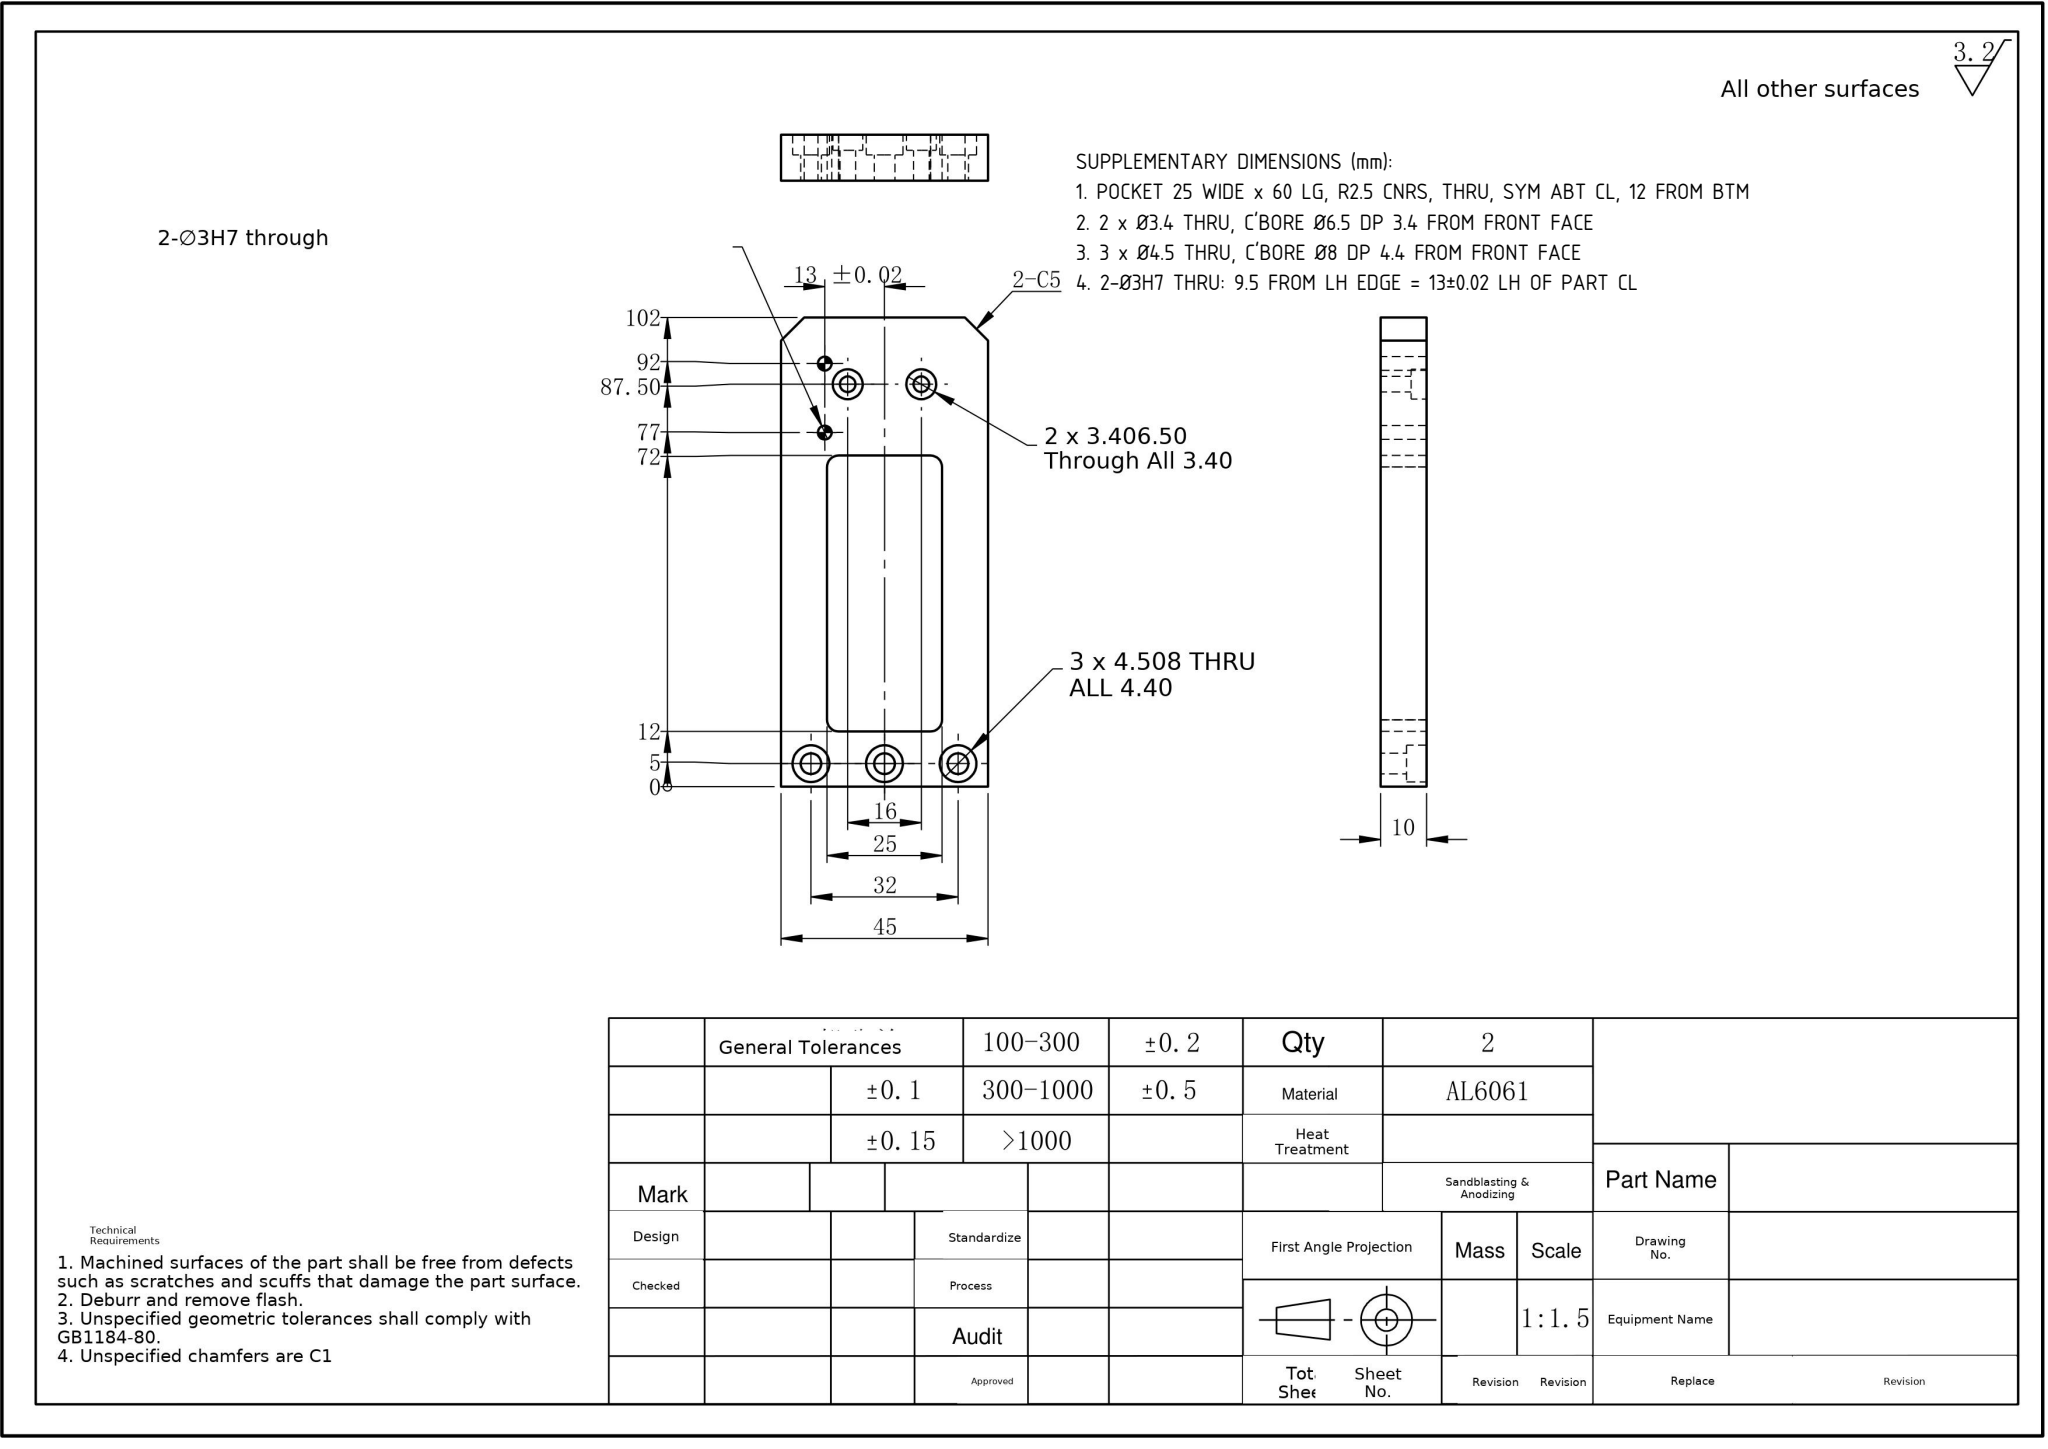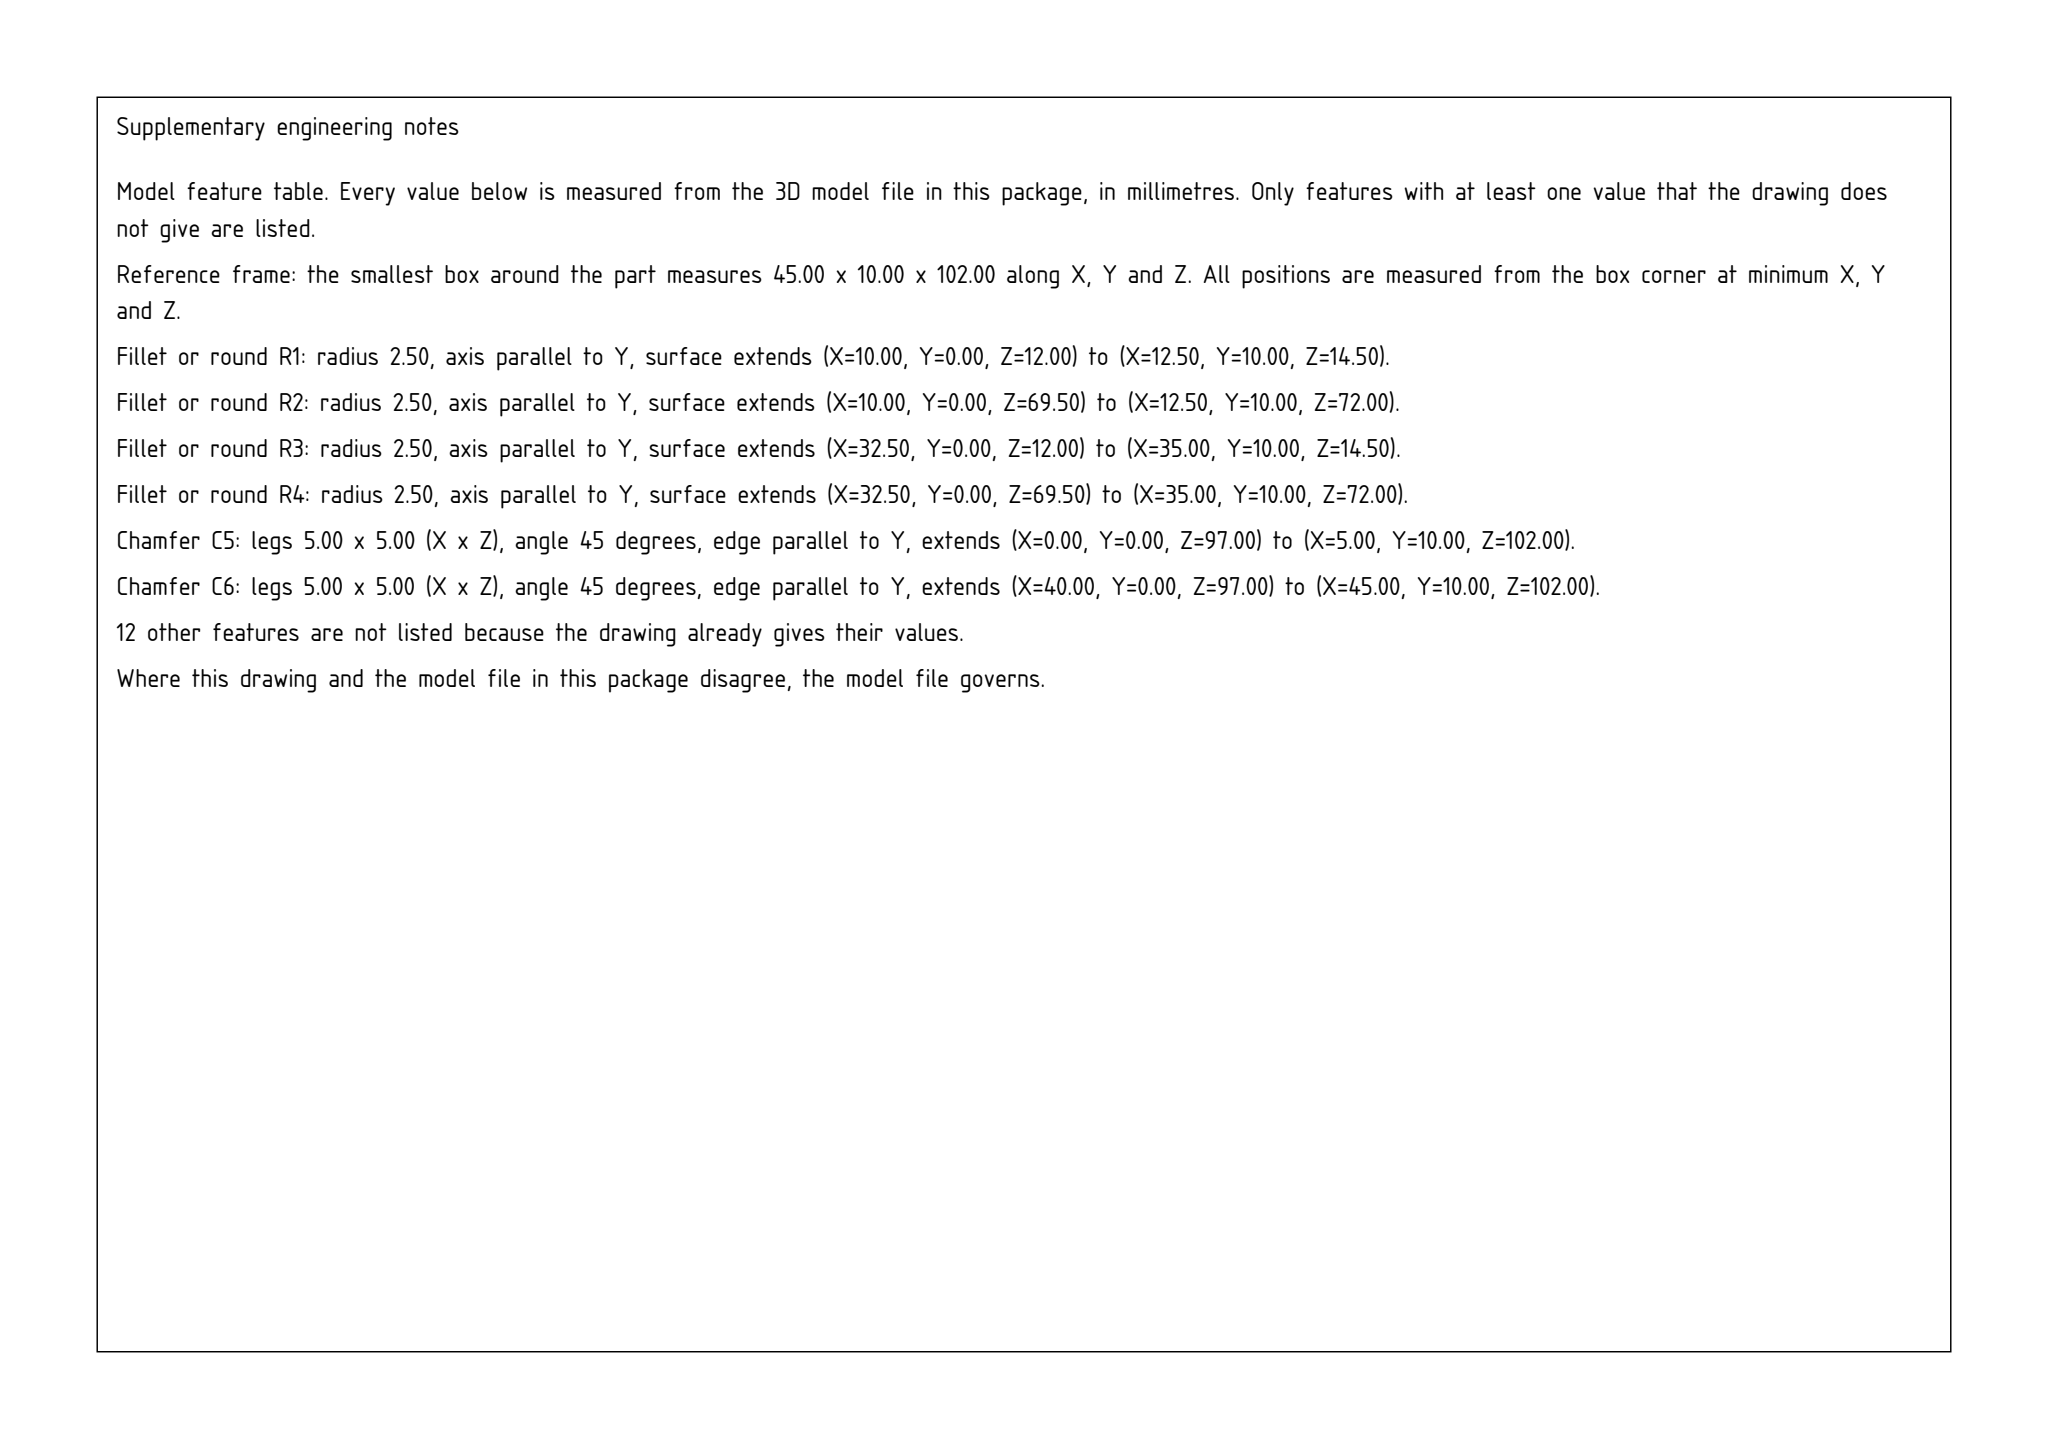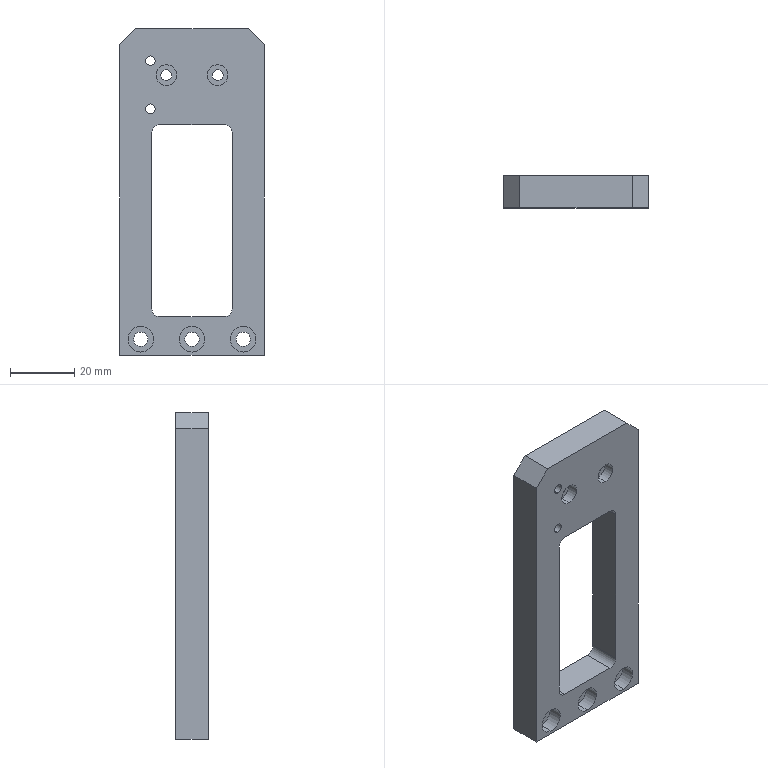Part | SolidWorks | mm | 1 solid | 45 faces | box 45 x 10 x 102 mm | volume 29286 mm3 | cylinder 28 | plane 17 | commonest cylinder face diameters 8 x6 4.5 x6 3 x4 6.5 x4 3.4 x4 5 x4
build123d program:
from build123d import *

# Parameters (mm, degrees)
SKETCH1_W                                       = 45
SKETCH1_H                                       = 102
BOSS_EXTRUDE1_DEPTH                             = 5
M4_HEX_SOCKET_HEAD_CAP_SCREW_CBORE1_D           = 4.5
M4_HEX_SOCKET_HEAD_CAP_SCREW_CBORE1_CBORE_D     = 8
M4_HEX_SOCKET_HEAD_CAP_SCREW_CBORE1_CBORE_DEPTH = 4.4
CHAMFER1_SIZE                                   = 5
M3_HEX_SOCKET_HEAD_CAP_SCREW_CBORE1_D           = 3.4
M3_HEX_SOCKET_HEAD_CAP_SCREW_CBORE1_CBORE_D     = 6.5
M3_HEX_SOCKET_HEAD_CAP_SCREW_CBORE1_CBORE_DEPTH = 3.4
SKETCH6_W                                       = 25
SKETCH6_H                                       = 60
CUT_EXTRUDE1_DEPTH                              = 10
FILLET1_R                                       = 2.5
SKETCH7_R                                       = 1.5
CUT_EXTRUDE2_DEPTH                              = 10


with BuildPart() as part:
    # Sketch1 → Boss-Extrude1 (new, symmetric)
    with BuildSketch(Plane(origin=(0, 0, 0), x_dir=(1, 0, 0), z_dir=(0, 1, 0))):
        Rectangle(SKETCH1_W, SKETCH1_H)
    extrude(amount=BOSS_EXTRUDE1_DEPTH, both=True)

    # M4 Hex Socket Head Cap Screw CBORE1 (through all)
    with Locations(Plane(origin=(0, -5, 0), x_dir=(-1, 0, 0), z_dir=(0, -1, 0))):
        with Locations((0, 46), (16, 46), (-16, 46)):
            CounterBoreHole(M4_HEX_SOCKET_HEAD_CAP_SCREW_CBORE1_D / 2, M4_HEX_SOCKET_HEAD_CAP_SCREW_CBORE1_CBORE_D / 2, M4_HEX_SOCKET_HEAD_CAP_SCREW_CBORE1_CBORE_DEPTH)

    # Chamfer1
    chamfer1_edges = [part.edges().sort_by_distance(p)[0] for p in [
        (22.5, 0, 51),
        (-22.5, 0, 51),
    ]]
    chamfer(chamfer1_edges, length=CHAMFER1_SIZE)

    # M3 Hex Socket Head Cap Screw CBORE1 (through all)
    with Locations(Plane(origin=(0, -5, 0), x_dir=(-1, 0, 0), z_dir=(0, -1, 0))):
        with Locations((-8, -36.5), (8, -36.5)):
            CounterBoreHole(M3_HEX_SOCKET_HEAD_CAP_SCREW_CBORE1_D / 2, M3_HEX_SOCKET_HEAD_CAP_SCREW_CBORE1_CBORE_D / 2, M3_HEX_SOCKET_HEAD_CAP_SCREW_CBORE1_CBORE_DEPTH)

    # Sketch6 → Cut-Extrude1 (cut)
    with BuildSketch(Plane(origin=(0, 5, 0), x_dir=(1, 0, 0), z_dir=(0, 1, 0))):
        with Locations((0, 9)):
            Rectangle(SKETCH6_W, SKETCH6_H)
    extrude(amount=-CUT_EXTRUDE1_DEPTH, mode=Mode.SUBTRACT)

    # Fillet1
    fillet1_edges = [part.edges().sort_by_distance(p)[0] for p in [
        (-12.5, 0, 21),
        (-12.5, 0, -39),
        (12.5, 0, -39),
        (12.5, 0, 21),
    ]]
    fillet(fillet1_edges, radius=FILLET1_R)

    # Sketch7 → Cut-Extrude2 (cut)
    with BuildSketch(Plane(origin=(0, 5, 0), x_dir=(1, 0, 0), z_dir=(0, 1, 0))):
        with Locations(Location((-13, -26, 0), (0, 0, 270))):
            Circle(SKETCH7_R)
        with Locations(Location((-13, -41, 0), (0, 0, 270))):
            Circle(SKETCH7_R)
    extrude(amount=-CUT_EXTRUDE2_DEPTH, mode=Mode.SUBTRACT)


solid = part.part